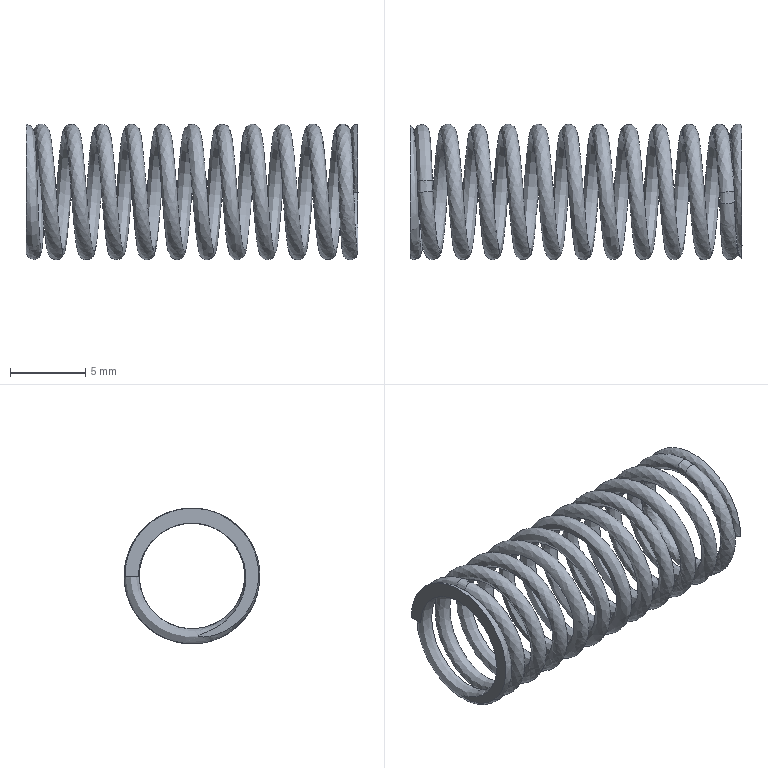Component | NX | SPRING_CYLINDER_COMPRESSION_1 | 1 solid | 9 faces | volume 236 mm3 | spline 5 | plane 4